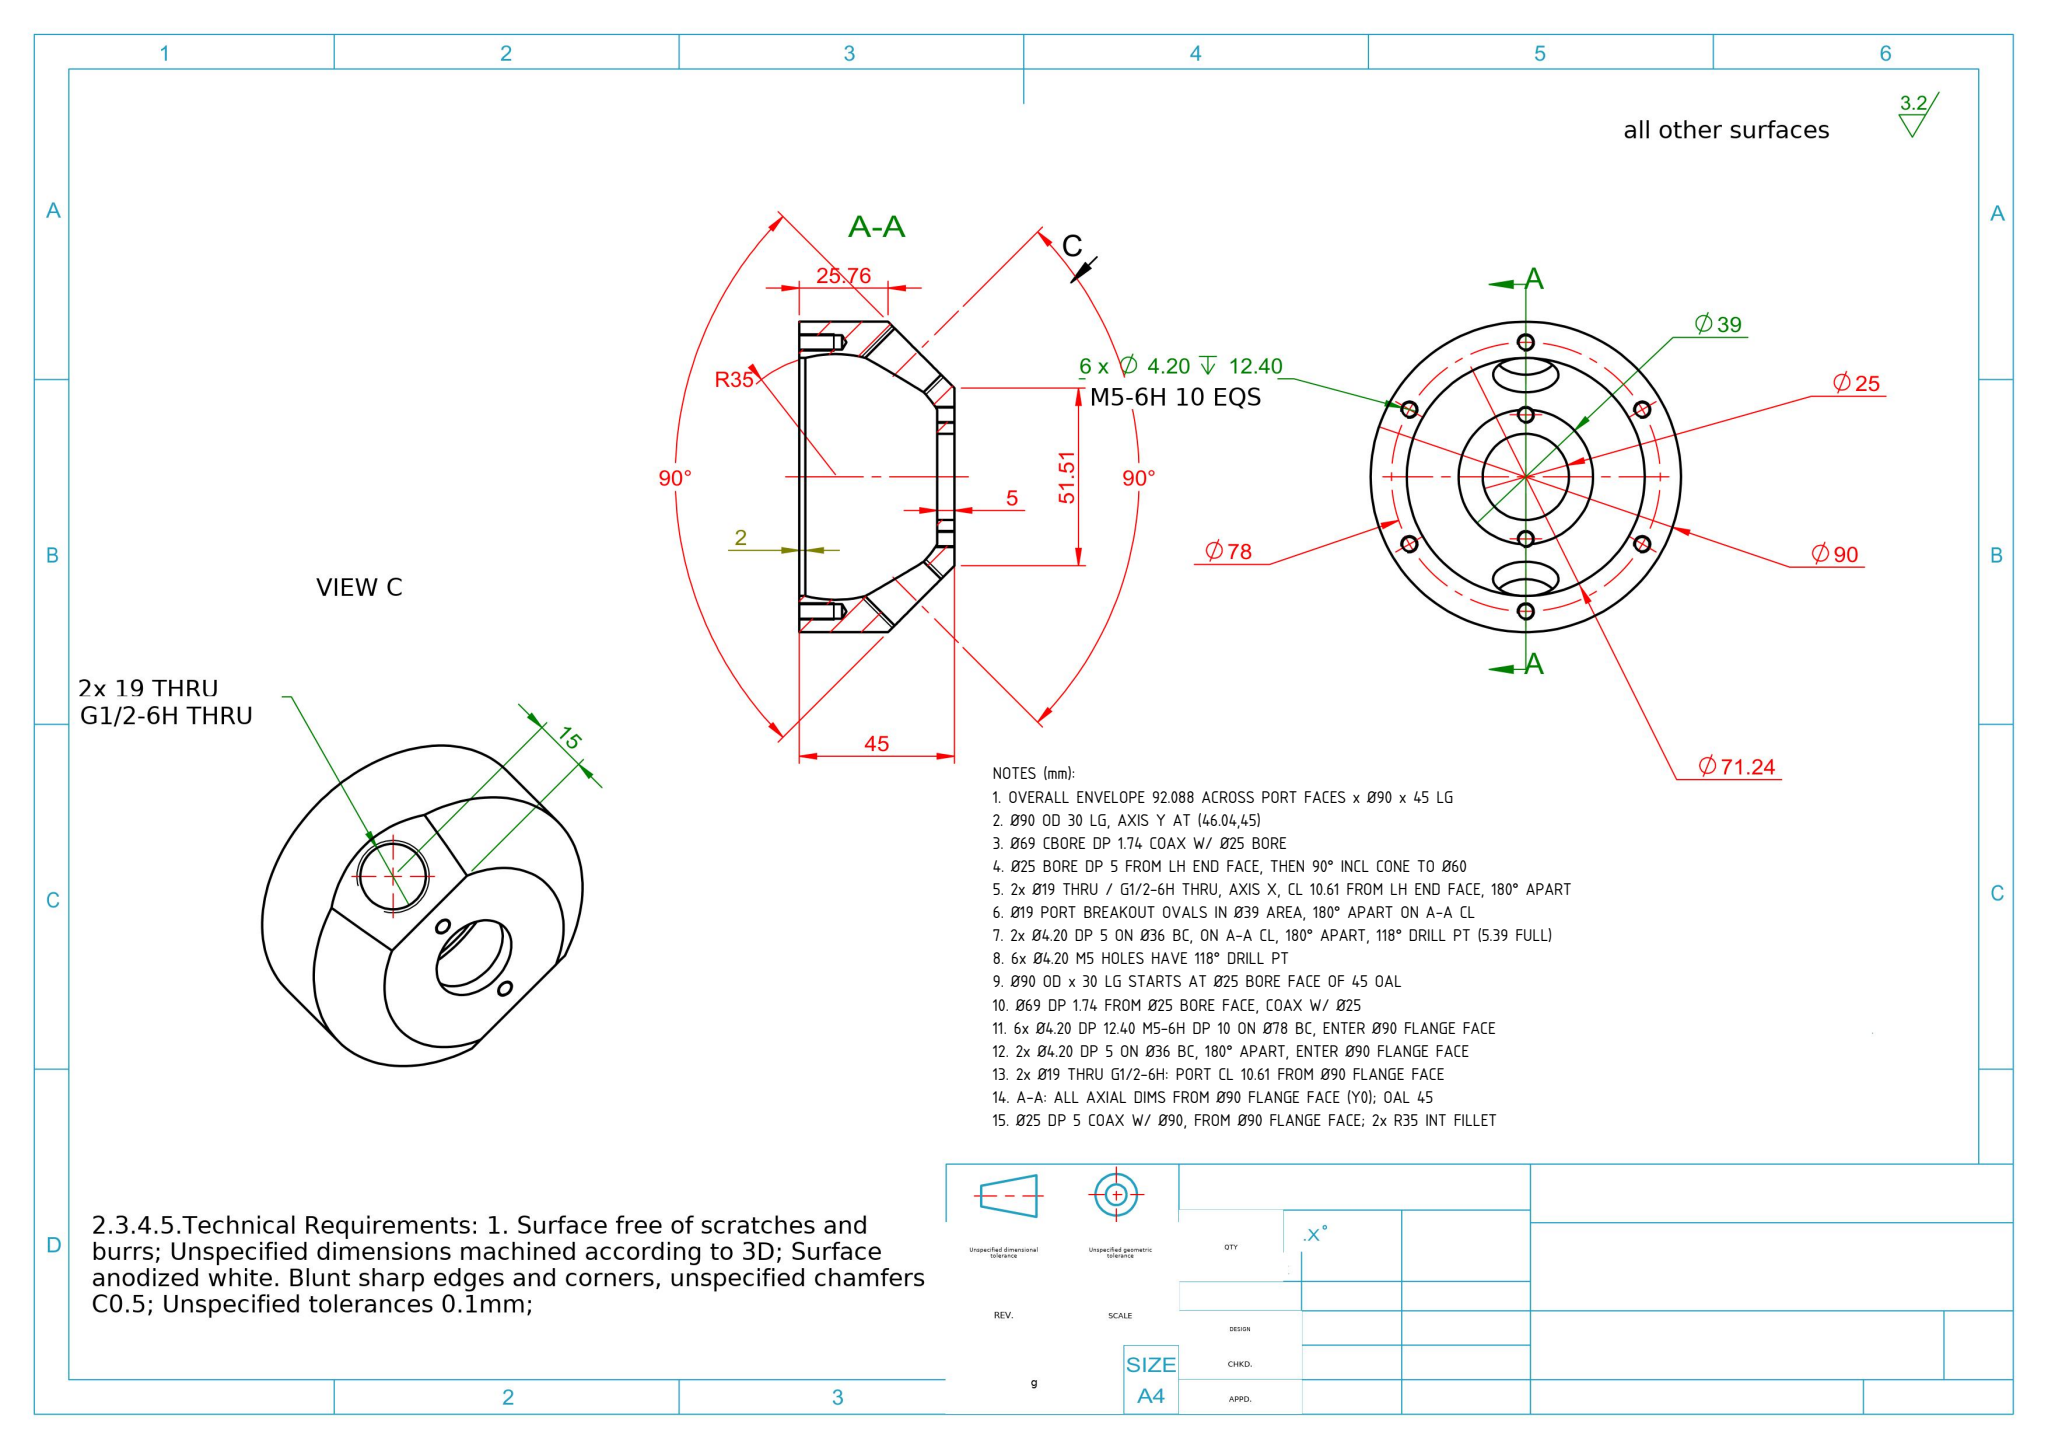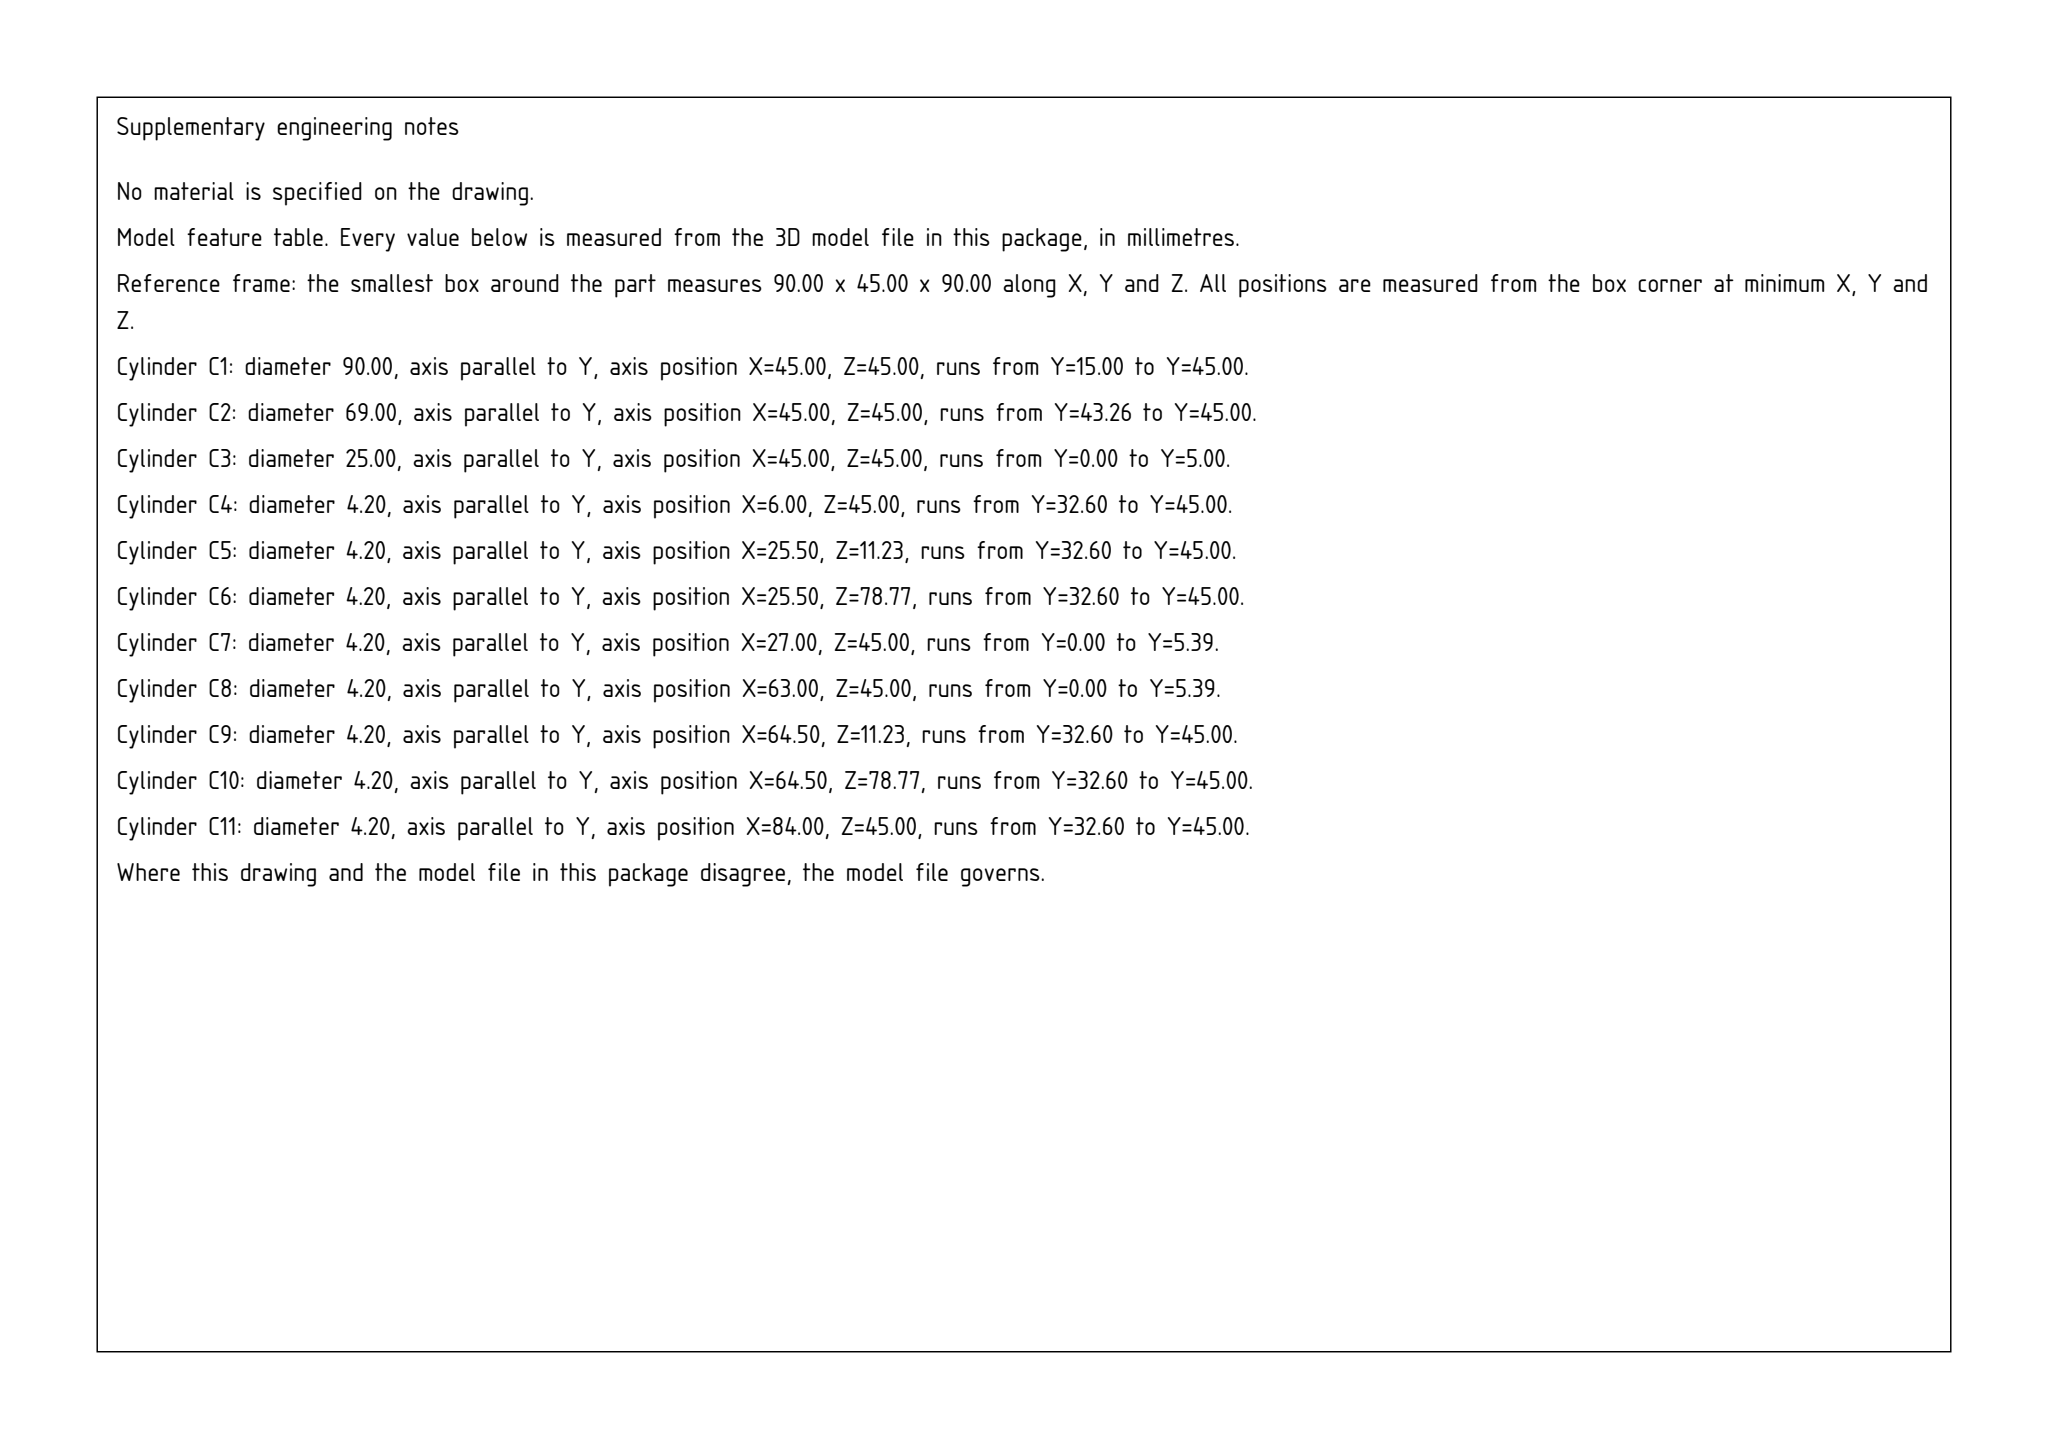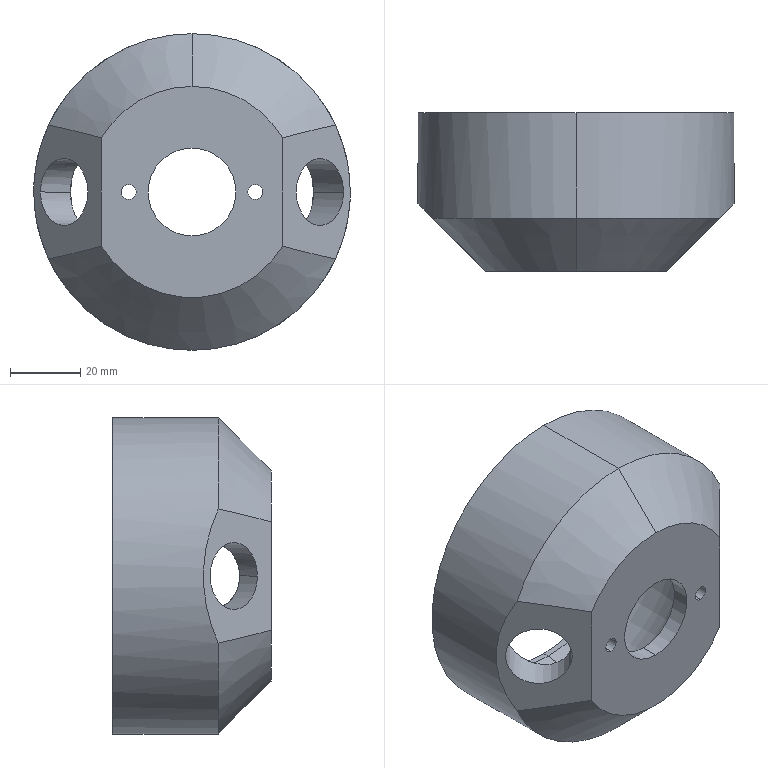Part | SolidWorks | mm | 1 solid | 48 faces | box 90 x 45 x 90 mm | volume 115037 mm3 | cylinder 26 | cone 15 | plane 5 | torus 2 | commonest cylinder face diameters 4.2 x16 19 x4 69 x2 25 x2 90 x2
Drawing notes:
OVERALL ENVELOPE 92.088 ACROSS PORT FACES x Ø90 x 45 LG | from the solid: bbox 92.088 x 45 x 90
Ø90 OD 30 LG, AXIS Y AT (46.04,45) | from the solid: Ø90 cyl, axis Y at (46.04,45), 30 lg
Ø69 CBORE DP 1.74 COAX W/ Ø25 BORE | from the solid: Ø69 cyl 1.74 lg, axis Y at (46.04,45)
Ø25 BORE DP 5 FROM LH END FACE, THEN 90° INCL CONE TO Ø60 | from the solid: Ø25 cyl 5.0 lg, axis Y at (46.04,45); planes y=0 and y=5; cone 90° incl, ref dia 60
2x Ø19 THRU / G1/2-6H THRU, AXIS X, CL 10.61 FROM LH END FACE, 180° APART | from the solid: two Ø19 cyls, axis X, y=10.61, z=45, 21.97 lg, one each end of 92.088 bbox
Ø19 PORT BREAKOUT OVALS IN Ø39 AREA, 180° APART ON A-A CL | from the solid: Ø19 X-axis holes break into 90° incl cone (ref Ø60) coaxial with Ø90
2x Ø4.20 DP 5 ON Ø36 BC, ON A-A CL, 180° APART, 118° DRILL PT (5.39 FULL) | from the solid: Ø4.2 Y-axis holes x=28.04 and x=64.04, z=45 (R18 from 46.04,45), 5.0 lg / 5.39 w/ pt
6x Ø4.20 M5 HOLES HAVE 118° DRILL PT | from the solid: cones 118° incl, ref dia 4.2, count 12
Ø90 OD x 30 LG STARTS AT Ø25 BORE FACE OF 45 OAL | from the solid: Ø90 y-axis cyl L=30 coax w/ Ø25 bore at x46.04 z45; y-planes at 0 and 45 give 45 OAL, Ø90 runs y0-30
Ø69 DP 1.74 FROM Ø25 BORE FACE, COAX W/ Ø25 | from the solid: Ø69 y-axis cyl L=1.74 at x46.04 z45, same face (y=0) as Ø25 x 5 DP bore
6x Ø4.20 DP 12.40 M5-6H DP 10 ON Ø78 BC, ENTER Ø90 FLANGE FACE | from the solid: Ø4.2 y-axis cyls L=12.40 at (7.04,45),(85.04,45),(26.54,11.23),(26.54,78.78),(65.54,11.23),(65.54,78.78) = R39 (Ø78 BC) about centre (46.04,45); start at y=0 flange face
2x Ø4.20 DP 5 ON Ø36 BC, 180° APART, ENTER Ø90 FLANGE FACE | from the solid: Ø4.2 y-axis cyls L=5.0 (5.39 w/118° point) at x=28.04 & 64.04, z=45, i.e. ±18 from centre 46.04 = Ø36 BC; start at y=0 face
2x Ø19 THRU G1/2-6H: PORT CL 10.61 FROM Ø90 FLANGE FACE | from the solid: Ø19 x-axis cyls, L=21.97, pos y=10.61, z=45 (part CL); bbox y=45 with faces at y=0/45
A-A: ALL AXIAL DIMS FROM Ø90 FLANGE FACE (Y0); OAL 45 | from the solid: planes normal y at 0.0, 5.0, 45.0; bbox Y=45; Ø90 cyl 30 lg from y=0
Ø25 DP 5 COAX W/ Ø90, FROM Ø90 FLANGE FACE; 2x R35 INT FILLET | from the solid: Ø25 y-axis cyl L=5.0 at (46.04,45) with plane y=5.0; fillet_radii 35.0 x2
build123d program:
from build123d import *

# Parameters (mm, degrees)
SKETCH13_W            = 111.106
SKETCH13_H            = 115.586
CUT_EXTRUDE3_DEPTH    = 3
G1_2_TAPPED_HOLE3_D   = 19
SKETCH16_R            = 34.5
CUT_EXTRUDE4_DEPTH    = 2
CIRPATTERN2_COUNT     = 6
M5_TAPPED_HOLE2_D     = 4.2
M5_TAPPED_HOLE2_DEPTH = 12.4
M5_TAPPED_HOLE2_TIP   = 1.262


with BuildPart() as part:
    # Sketch5 → Revolve1 (revolve)
    with BuildSketch(Plane.XY, mode=Mode.PRIVATE) as revolve1_sk:
        with BuildLine():
            Line((12.5, 0), (30, 0))
            Line((30, 0), (45, 15))
            Line((45, 15), (45, 45))
            Line((45, 45), (34, 45))
            ThreePointArc((34, 45), (33.526, 22.544), (19.5, 5))
            Line((19.5, 5), (12.5, 5))
            Line((12.5, 5), (12.5, 0))
        make_face()
    revolve(revolve1_sk.sketch.rotate(Axis((0, 0, 0), (0, 1, 0)), 90), axis=Axis((0, 0, 0), (0, 1, 0)))

    # Sketch13 → Cut-Extrude3 (cut)
    with BuildSketch(Plane(origin=(-15, -15, 0), x_dir=(0, 0, 1), z_dir=(-0.7071, -0.7071, 0))):
        with Locations((6.284, 19.659)):
            Rectangle(SKETCH13_W, SKETCH13_H)
    cut_extrude3 = extrude(amount=-CUT_EXTRUDE3_DEPTH, mode=Mode.SUBTRACT)

    # G1_2 Tapped Hole3 (through all)
    with Locations(Plane(origin=(-12.879, -12.879, 0), x_dir=(0, 0, 1), z_dir=(-0.7071, -0.7071, 0))):
        with Locations((0, 33.213)):
            g1_2_tapped_hole3 = Hole(G1_2_TAPPED_HOLE3_D / 2)

    # Mirror3: Cut-Extrude3, G1_2 Tapped Hole3 across plane
    add(cut_extrude3.mirror(Plane(origin=(0, 0, 0), x_dir=(0, 0, 1), z_dir=(1, 0, 0))), mode=Mode.SUBTRACT)
    add(g1_2_tapped_hole3.mirror(Plane(origin=(0, 0, 0), x_dir=(0, 0, 1), z_dir=(1, 0, 0))), mode=Mode.SUBTRACT)

    # Sketch16 → Cut-Extrude4 (cut)
    with BuildSketch(Plane(origin=(0, 45, 0), x_dir=(1, 0, 0), z_dir=(0, 1, 0))):
        with Locations(Location((0, 0, 0), (0, 0, 270))):
            Circle(SKETCH16_R)
    extrude(amount=-CUT_EXTRUDE4_DEPTH, mode=Mode.SUBTRACT)

    # Sketch21 → M5 Tapped Hole1 (revolve, cut)
    with BuildSketch(Plane(origin=(-39, 45, 0), x_dir=(0, 0, 1), z_dir=(1, 0, 0))):
        Polygon((0, 0), (0, 13.662), (2.1, 12.4), (2.1, 0), align=None)
    m5_tapped_hole1 = revolve(axis=Axis((-39, 51.35, 0), (0, -1, 0)), mode=Mode.SUBTRACT)

    # CirPattern2: M5 Tapped Hole1 ×6 about axis
    cirpattern2_axis = Axis((0, 0, 0), (0, 1, 0))
    for i in range(1, CIRPATTERN2_COUNT):
        add(m5_tapped_hole1.rotate(cirpattern2_axis, i * 360 / CIRPATTERN2_COUNT), mode=Mode.SUBTRACT)

    # M5 Tapped Hole2
    with Locations(Plane(origin=(0, 0, 0), x_dir=(-1, 0, 0), z_dir=(0, -1, 0))):
        with Locations((-18, 0), (18, 0)):
            Hole(M5_TAPPED_HOLE2_D / 2, depth=M5_TAPPED_HOLE2_DEPTH)
            with Locations((0, 0, -(M5_TAPPED_HOLE2_DEPTH + M5_TAPPED_HOLE2_TIP / 2))):  # 118° drill point
                Cone(0, M5_TAPPED_HOLE2_D / 2, M5_TAPPED_HOLE2_TIP, mode=Mode.SUBTRACT)


solid = part.part